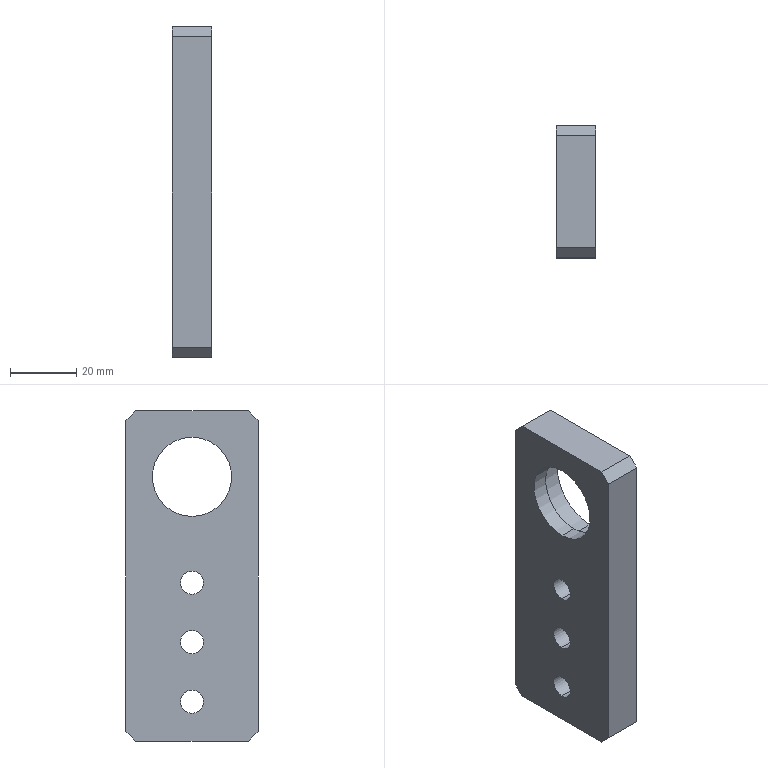Component | SolidWorks | ConveyorDriveWheelSidePlate-3 | 1 solid | 21 faces | box 12 x 40 x 100 mm | volume 39826 mm3 | plane 11 | cylinder 10 | commonest cylinder face diameters 7 x6 24 x2 28 x2 | material Plain Carbon Steel
build123d program:
from build123d import *

# Parameters (mm, degrees)
SKETCH1_W           = 100
SKETCH1_H           = 40
BOSS_EXTRUDE1_DEPTH = 12
SKETCH2_R           = 14
CUT_EXTRUDE1_DEPTH  = 7
SKETCH3_R           = 3.5
CUT_EXTRUDE2_DEPTH  = 56.172
SKETCH4_R           = 12
CUT_EXTRUDE3_DEPTH  = 55.305
CHAMFER1_SIZE       = 3


with BuildPart() as part:
    # Sketch1 → Boss-Extrude1 (new body)
    with BuildSketch(Plane(origin=(0, 0, 0), x_dir=(0, 0, -1), z_dir=(1, 0, 0))):
        Rectangle(SKETCH1_W, SKETCH1_H)
    extrude(amount=BOSS_EXTRUDE1_DEPTH)

    # Sketch2 → Cut-Extrude1 (cut)
    with BuildSketch(Plane(origin=(12, 0, 0), x_dir=(0, 0, -1), z_dir=(1, 0, 0))):
        with Locations((30, 0)):
            Circle(SKETCH2_R)
    extrude(amount=-CUT_EXTRUDE1_DEPTH, mode=Mode.SUBTRACT)

    # Sketch3 → Cut-Extrude2 (cut, through all)
    with BuildSketch(Plane.ZY):
        with Locations((38, 0)):
            Circle(SKETCH3_R)
        with Locations((2, 0)):
            Circle(SKETCH3_R)
        with Locations((20, 0)):
            Circle(SKETCH3_R)
    extrude(amount=-CUT_EXTRUDE2_DEPTH, mode=Mode.SUBTRACT)

    # Sketch4 → Cut-Extrude3 (cut, through all)
    with BuildSketch(Plane(origin=(5, 0, 0), x_dir=(0, 0, -1), z_dir=(1, 0, 0))):
        with Locations((30, 0)):
            Circle(SKETCH4_R)
    extrude(amount=-CUT_EXTRUDE3_DEPTH, mode=Mode.SUBTRACT)

    # Chamfer1
    chamfer1_edges = [part.edges().sort_by_distance(p)[0] for p in [
        (6, -20, -50),
        (6, -20, 50),
        (6, 20, 50),
        (6, 20, -50),
    ]]
    chamfer(chamfer1_edges, length=CHAMFER1_SIZE)


solid = part.part

# Placed as in the assembly
solid = solid.moved(Location((35.45, 5.646, 1505), (180, 0, 0)))
STEP:
#1=COLOUR_RGB('',0.7922,0.8196,0.9333);
#2=FILL_AREA_STYLE_COLOUR('',#1);
#3=FILL_AREA_STYLE('',(#2));
#4=SURFACE_STYLE_FILL_AREA(#3);
#5=SURFACE_SIDE_STYLE('',(#4));
#6=SURFACE_STYLE_USAGE(.BOTH.,#5);
#7=PRESENTATION_STYLE_ASSIGNMENT((#6));
#8=CARTESIAN_POINT('',(1.396,0.2223,59.961));
#9=VERTEX_POINT('',#8);
#10=CARTESIAN_POINT('',(1.396,0.2223,60.906));
#11=VERTEX_POINT('',#10);
#12=CARTESIAN_POINT('',(1.396,0.2223,60.433));
#13=DIRECTION('',(1.,-0.,-0.));
#14=DIRECTION('',(0.,0.,1.));
#15=AXIS2_PLACEMENT_3D('',#12,#13,#14);
#16=CIRCLE('',#15,0.4724);
#17=EDGE_CURVE('',#9,#11,#16,.T.);
#18=ORIENTED_EDGE('',*,*,#17,.F.);
#19=CARTESIAN_POINT('',(1.593,0.2223,59.961));
#20=VERTEX_POINT('',#19);
#21=CARTESIAN_POINT('',(1.396,0.2223,59.961));
#22=DIRECTION('',(1.,-0.,-0.));
#23=VECTOR('',#22,39.37);
#24=LINE('',#21,#23);
#25=EDGE_CURVE('',#9,#20,#24,.T.);
#26=ORIENTED_EDGE('',*,*,#25,.T.);
#27=CARTESIAN_POINT('',(1.593,0.2223,60.906));
#28=VERTEX_POINT('',#27);
#29=CARTESIAN_POINT('',(1.593,0.2223,60.433));
#30=DIRECTION('',(1.,-0.,-0.));
#31=DIRECTION('',(0.,0.,1.));
#32=AXIS2_PLACEMENT_3D('',#29,#30,#31);
#33=CIRCLE('',#32,0.4724);
#34=EDGE_CURVE('',#20,#28,#33,.T.);
#35=ORIENTED_EDGE('',*,*,#34,.T.);
#36=CARTESIAN_POINT('',(1.396,0.2223,60.906));
#37=DIRECTION('',(1.,-0.,-0.));
#38=VECTOR('',#37,39.37);
#39=LINE('',#36,#38);
#40=EDGE_CURVE('',#11,#28,#39,.T.);
#41=ORIENTED_EDGE('',*,*,#40,.F.);
#42=EDGE_LOOP('',(#18,#26,#35,#41));
#43=FACE_OUTER_BOUND('',#42,.T.);
#44=CARTESIAN_POINT('',(1.396,0.2223,60.433));
#45=DIRECTION('',(1.,-0.,-0.));
#46=DIRECTION('',(0.,0.,1.));
#47=AXIS2_PLACEMENT_3D('',#44,#45,#46);
#48=CYLINDRICAL_SURFACE('',#47,0.4724);
#49=ADVANCED_FACE('',(#43),#48,.F.);
#50=CARTESIAN_POINT('',(1.868,0.2223,58.602));
#51=VERTEX_POINT('',#50);
#52=CARTESIAN_POINT('',(1.868,0.2223,58.327));
#53=VERTEX_POINT('',#52);
#54=CARTESIAN_POINT('',(1.868,0.2223,58.465));
#55=DIRECTION('',(-1.,0.,0.));
#56=DIRECTION('',(0.,0.,-1.));
#57=AXIS2_PLACEMENT_3D('',#54,#55,#56);
#58=CIRCLE('',#57,0.1378);
#59=EDGE_CURVE('',#51,#53,#58,.T.);
#60=ORIENTED_EDGE('',*,*,#59,.F.);
#61=CARTESIAN_POINT('',(1.396,0.2223,58.602));
#62=VERTEX_POINT('',#61);
#63=CARTESIAN_POINT('',(1.868,0.2223,58.602));
#64=DIRECTION('',(-1.,0.,0.));
#65=VECTOR('',#64,39.37);
#66=LINE('',#63,#65);
#67=EDGE_CURVE('',#51,#62,#66,.T.);
#68=ORIENTED_EDGE('',*,*,#67,.T.);
#69=CARTESIAN_POINT('',(1.396,0.2223,58.327));
#70=VERTEX_POINT('',#69);
#71=CARTESIAN_POINT('',(1.396,0.2223,58.465));
#72=DIRECTION('',(-1.,0.,0.));
#73=DIRECTION('',(0.,0.,-1.));
#74=AXIS2_PLACEMENT_3D('',#71,#72,#73);
#75=CIRCLE('',#74,0.1378);
#76=EDGE_CURVE('',#62,#70,#75,.T.);
#77=ORIENTED_EDGE('',*,*,#76,.T.);
#78=CARTESIAN_POINT('',(1.868,0.2223,58.327));
#79=DIRECTION('',(-1.,0.,0.));
#80=VECTOR('',#79,39.37);
#81=LINE('',#78,#80);
#82=EDGE_CURVE('',#53,#70,#81,.T.);
#83=ORIENTED_EDGE('',*,*,#82,.F.);
#84=EDGE_LOOP('',(#60,#68,#77,#83));
#85=FACE_OUTER_BOUND('',#84,.T.);
#86=CARTESIAN_POINT('',(1.868,0.2223,58.465));
#87=DIRECTION('',(-1.,0.,0.));
#88=DIRECTION('',(0.,0.,-1.));
#89=AXIS2_PLACEMENT_3D('',#86,#87,#88);
#90=CYLINDRICAL_SURFACE('',#89,0.1378);
#91=ADVANCED_FACE('',(#85),#90,.F.);
#92=CARTESIAN_POINT('',(1.868,0.2223,59.311));
#93=VERTEX_POINT('',#92);
#94=CARTESIAN_POINT('',(1.868,0.2223,59.035));
#95=VERTEX_POINT('',#94);
#96=CARTESIAN_POINT('',(1.868,0.2223,59.173));
#97=DIRECTION('',(-1.,0.,0.));
#98=DIRECTION('',(0.,0.,-1.));
#99=AXIS2_PLACEMENT_3D('',#96,#97,#98);
#100=CIRCLE('',#99,0.1378);
#101=EDGE_CURVE('',#93,#95,#100,.T.);
#102=ORIENTED_EDGE('',*,*,#101,.F.);
#103=CARTESIAN_POINT('',(1.396,0.2223,59.311));
#104=VERTEX_POINT('',#103);
#105=CARTESIAN_POINT('',(1.868,0.2223,59.311));
#106=DIRECTION('',(-1.,0.,0.));
#107=VECTOR('',#106,39.37);
#108=LINE('',#105,#107);
#109=EDGE_CURVE('',#93,#104,#108,.T.);
#110=ORIENTED_EDGE('',*,*,#109,.T.);
#111=CARTESIAN_POINT('',(1.396,0.2223,59.035));
#112=VERTEX_POINT('',#111);
#113=CARTESIAN_POINT('',(1.396,0.2223,59.173));
#114=DIRECTION('',(-1.,0.,0.));
#115=DIRECTION('',(0.,0.,-1.));
#116=AXIS2_PLACEMENT_3D('',#113,#114,#115);
#117=CIRCLE('',#116,0.1378);
#118=EDGE_CURVE('',#104,#112,#117,.T.);
#119=ORIENTED_EDGE('',*,*,#118,.T.);
#120=CARTESIAN_POINT('',(1.868,0.2223,59.035));
#121=DIRECTION('',(-1.,0.,0.));
#122=VECTOR('',#121,39.37);
#123=LINE('',#120,#122);
#124=EDGE_CURVE('',#95,#112,#123,.T.);
#125=ORIENTED_EDGE('',*,*,#124,.F.);
#126=EDGE_LOOP('',(#102,#110,#119,#125));
#127=FACE_OUTER_BOUND('',#126,.T.);
#128=CARTESIAN_POINT('',(1.868,0.2223,59.173));
#129=DIRECTION('',(-1.,0.,0.));
#130=DIRECTION('',(0.,0.,-1.));
#131=AXIS2_PLACEMENT_3D('',#128,#129,#130);
#132=CYLINDRICAL_SURFACE('',#131,0.1378);
#133=ADVANCED_FACE('',(#127),#132,.F.);
#134=CARTESIAN_POINT('',(1.868,0.2223,57.894));
#135=VERTEX_POINT('',#134);
#136=CARTESIAN_POINT('',(1.868,0.2223,57.618));
#137=VERTEX_POINT('',#136);
#138=CARTESIAN_POINT('',(1.868,0.2223,57.756));
#139=DIRECTION('',(-1.,0.,0.));
#140=DIRECTION('',(0.,0.,-1.));
#141=AXIS2_PLACEMENT_3D('',#138,#139,#140);
#142=CIRCLE('',#141,0.1378);
#143=EDGE_CURVE('',#135,#137,#142,.T.);
#144=ORIENTED_EDGE('',*,*,#143,.F.);
#145=CARTESIAN_POINT('',(1.396,0.2223,57.894));
#146=VERTEX_POINT('',#145);
#147=CARTESIAN_POINT('',(1.868,0.2223,57.894));
#148=DIRECTION('',(-1.,0.,0.));
#149=VECTOR('',#148,39.37);
#150=LINE('',#147,#149);
#151=EDGE_CURVE('',#135,#146,#150,.T.);
#152=ORIENTED_EDGE('',*,*,#151,.T.);
#153=CARTESIAN_POINT('',(1.396,0.2223,57.618));
#154=VERTEX_POINT('',#153);
#155=CARTESIAN_POINT('',(1.396,0.2223,57.756));
#156=DIRECTION('',(-1.,0.,0.));
#157=DIRECTION('',(0.,0.,-1.));
#158=AXIS2_PLACEMENT_3D('',#155,#156,#157);
#159=CIRCLE('',#158,0.1378);
#160=EDGE_CURVE('',#146,#154,#159,.T.);
#161=ORIENTED_EDGE('',*,*,#160,.T.);
#162=CARTESIAN_POINT('',(1.868,0.2223,57.618));
#163=DIRECTION('',(-1.,0.,0.));
#164=VECTOR('',#163,39.37);
#165=LINE('',#162,#164);
#166=EDGE_CURVE('',#137,#154,#165,.T.);
#167=ORIENTED_EDGE('',*,*,#166,.F.);
#168=EDGE_LOOP('',(#144,#152,#161,#167));
#169=FACE_OUTER_BOUND('',#168,.T.);
#170=CARTESIAN_POINT('',(1.868,0.2223,57.756));
#171=DIRECTION('',(-1.,0.,0.));
#172=DIRECTION('',(0.,0.,-1.));
#173=AXIS2_PLACEMENT_3D('',#170,#171,#172);
#174=CYLINDRICAL_SURFACE('',#173,0.1378);
#175=ADVANCED_FACE('',(#169),#174,.F.);
#176=CARTESIAN_POINT('',(1.593,0.2223,59.882));
#177=VERTEX_POINT('',#176);
#178=CARTESIAN_POINT('',(1.593,0.2223,60.984));
#179=VERTEX_POINT('',#178);
#180=CARTESIAN_POINT('',(1.593,0.2223,60.433));
#181=DIRECTION('',(1.,-0.,-0.));
#182=DIRECTION('',(0.,0.,1.));
#183=AXIS2_PLACEMENT_3D('',#180,#181,#182);
#184=CIRCLE('',#183,0.5512);
#185=EDGE_CURVE('',#177,#179,#184,.T.);
#186=ORIENTED_EDGE('',*,*,#185,.F.);
#187=CARTESIAN_POINT('',(1.868,0.2223,59.882));
#188=VERTEX_POINT('',#187);
#189=CARTESIAN_POINT('',(1.593,0.2223,59.882));
#190=DIRECTION('',(1.,-0.,-0.));
#191=VECTOR('',#190,39.37);
#192=LINE('',#189,#191);
#193=EDGE_CURVE('',#177,#188,#192,.T.);
#194=ORIENTED_EDGE('',*,*,#193,.T.);
#195=CARTESIAN_POINT('',(1.868,0.2223,60.984));
#196=VERTEX_POINT('',#195);
#197=CARTESIAN_POINT('',(1.868,0.2223,60.433));
#198=DIRECTION('',(1.,-0.,-0.));
#199=DIRECTION('',(0.,0.,1.));
#200=AXIS2_PLACEMENT_3D('',#197,#198,#199);
#201=CIRCLE('',#200,0.5512);
#202=EDGE_CURVE('',#188,#196,#201,.T.);
#203=ORIENTED_EDGE('',*,*,#202,.T.);
#204=CARTESIAN_POINT('',(1.593,0.2223,60.984));
#205=DIRECTION('',(1.,-0.,-0.));
#206=VECTOR('',#205,39.37);
#207=LINE('',#204,#206);
#208=EDGE_CURVE('',#179,#196,#207,.T.);
#209=ORIENTED_EDGE('',*,*,#208,.F.);
#210=EDGE_LOOP('',(#186,#194,#203,#209));
#211=FACE_OUTER_BOUND('',#210,.T.);
#212=CARTESIAN_POINT('',(1.593,0.2223,60.433));
#213=DIRECTION('',(1.,-0.,-0.));
#214=DIRECTION('',(0.,0.,1.));
#215=AXIS2_PLACEMENT_3D('',#212,#213,#214);
#216=CYLINDRICAL_SURFACE('',#215,0.5512);
#217=ADVANCED_FACE('',(#211),#216,.F.);
#218=CARTESIAN_POINT('',(1.868,0.8916,61.22));
#219=VERTEX_POINT('',#218);
#220=CARTESIAN_POINT('',(1.868,-0.447,61.22));
#221=VERTEX_POINT('',#220);
#222=CARTESIAN_POINT('',(1.868,1.01,61.22));
#223=DIRECTION('',(-0.,-1.,0.));
#224=VECTOR('',#223,39.37);
#225=LINE('',#222,#224);
#226=EDGE_CURVE('',#219,#221,#225,.T.);
#227=ORIENTED_EDGE('',*,*,#226,.F.);
#228=CARTESIAN_POINT('',(1.396,0.8916,61.22));
#229=VERTEX_POINT('',#228);
#230=CARTESIAN_POINT('',(1.868,0.8916,61.22));
#231=DIRECTION('',(-1.,0.,0.));
#232=VECTOR('',#231,39.37);
#233=LINE('',#230,#232);
#234=EDGE_CURVE('',#219,#229,#233,.T.);
#235=ORIENTED_EDGE('',*,*,#234,.T.);
#236=CARTESIAN_POINT('',(1.396,-0.447,61.22));
#237=VERTEX_POINT('',#236);
#238=CARTESIAN_POINT('',(1.396,1.01,61.22));
#239=DIRECTION('',(-0.,-1.,0.));
#240=VECTOR('',#239,39.37);
#241=LINE('',#238,#240);
#242=EDGE_CURVE('',#229,#237,#241,.T.);
#243=ORIENTED_EDGE('',*,*,#242,.T.);
#244=CARTESIAN_POINT('',(1.868,-0.447,61.22));
#245=DIRECTION('',(1.,-0.,-0.));
#246=VECTOR('',#245,39.37);
#247=LINE('',#244,#246);
#248=EDGE_CURVE('',#237,#221,#247,.T.);
#249=ORIENTED_EDGE('',*,*,#248,.T.);
#250=EDGE_LOOP('',(#227,#235,#243,#249));
#251=FACE_OUTER_BOUND('',#250,.T.);
#252=CARTESIAN_POINT('',(1.868,1.01,61.22));
#253=DIRECTION('',(-0.,-0.,-1.));
#254=DIRECTION('',(1.,-0.,-0.));
#255=AXIS2_PLACEMENT_3D('',#252,#253,#254);
#256=PLANE('',#255);
#257=ADVANCED_FACE('',(#251),#256,.F.);
#258=CARTESIAN_POINT('',(1.868,-0.5651,61.102));
#259=VERTEX_POINT('',#258);
#260=CARTESIAN_POINT('',(1.868,-0.5651,57.402));
#261=VERTEX_POINT('',#260);
#262=CARTESIAN_POINT('',(1.868,-0.5651,57.283));
#263=DIRECTION('',(-0.,0.,-1.));
#264=VECTOR('',#263,39.37);
#265=LINE('',#262,#264);
#266=EDGE_CURVE('',#259,#261,#265,.T.);
#267=ORIENTED_EDGE('',*,*,#266,.F.);
#268=CARTESIAN_POINT('',(1.396,-0.5651,61.102));
#269=VERTEX_POINT('',#268);
#270=CARTESIAN_POINT('',(1.868,-0.5651,61.102));
#271=DIRECTION('',(-1.,0.,0.));
#272=VECTOR('',#271,39.37);
#273=LINE('',#270,#272);
#274=EDGE_CURVE('',#259,#269,#273,.T.);
#275=ORIENTED_EDGE('',*,*,#274,.T.);
#276=CARTESIAN_POINT('',(1.396,-0.5651,57.402));
#277=VERTEX_POINT('',#276);
#278=CARTESIAN_POINT('',(1.396,-0.5651,57.283));
#279=DIRECTION('',(-0.,0.,-1.));
#280=VECTOR('',#279,39.37);
#281=LINE('',#278,#280);
#282=EDGE_CURVE('',#269,#277,#281,.T.);
#283=ORIENTED_EDGE('',*,*,#282,.T.);
#284=CARTESIAN_POINT('',(1.868,-0.5651,57.402));
#285=DIRECTION('',(1.,-0.,-0.));
#286=VECTOR('',#285,39.37);
#287=LINE('',#284,#286);
#288=EDGE_CURVE('',#277,#261,#287,.T.);
#289=ORIENTED_EDGE('',*,*,#288,.T.);
#290=EDGE_LOOP('',(#267,#275,#283,#289));
#291=FACE_OUTER_BOUND('',#290,.T.);
#292=CARTESIAN_POINT('',(1.868,-0.5651,57.283));
#293=DIRECTION('',(0.,1.,-0.));
#294=DIRECTION('',(0.,0.,1.));
#295=AXIS2_PLACEMENT_3D('',#292,#293,#294);
#296=PLANE('',#295);
#297=ADVANCED_FACE('',(#291),#296,.F.);
#298=CARTESIAN_POINT('',(1.396,-0.447,57.283));
#299=VERTEX_POINT('',#298);
#300=CARTESIAN_POINT('',(1.396,0.8916,57.283));
#301=VERTEX_POINT('',#300);
#302=CARTESIAN_POINT('',(1.396,1.01,57.283));
#303=DIRECTION('',(0.,1.,-0.));
#304=VECTOR('',#303,39.37);
#305=LINE('',#302,#304);
#306=EDGE_CURVE('',#299,#301,#305,.T.);
#307=ORIENTED_EDGE('',*,*,#306,.T.);
#308=CARTESIAN_POINT('',(1.868,0.8916,57.283));
#309=VERTEX_POINT('',#308);
#310=CARTESIAN_POINT('',(1.868,0.8916,57.283));
#311=DIRECTION('',(1.,-0.,-0.));
#312=VECTOR('',#311,39.37);
#313=LINE('',#310,#312);
#314=EDGE_CURVE('',#301,#309,#313,.T.);
#315=ORIENTED_EDGE('',*,*,#314,.T.);
#316=CARTESIAN_POINT('',(1.868,-0.447,57.283));
#317=VERTEX_POINT('',#316);
#318=CARTESIAN_POINT('',(1.868,1.01,57.283));
#319=DIRECTION('',(0.,1.,-0.));
#320=VECTOR('',#319,39.37);
#321=LINE('',#318,#320);
#322=EDGE_CURVE('',#317,#309,#321,.T.);
#323=ORIENTED_EDGE('',*,*,#322,.F.);
#324=CARTESIAN_POINT('',(1.868,-0.447,57.283));
#325=DIRECTION('',(-1.,0.,0.));
#326=VECTOR('',#325,39.37);
#327=LINE('',#324,#326);
#328=EDGE_CURVE('',#317,#299,#327,.T.);
#329=ORIENTED_EDGE('',*,*,#328,.T.);
#330=EDGE_LOOP('',(#307,#315,#323,#329));
#331=FACE_OUTER_BOUND('',#330,.T.);
#332=CARTESIAN_POINT('',(1.868,1.01,57.283));
#333=DIRECTION('',(0.,0.,1.));
#334=DIRECTION('',(-1.,0.,0.));
#335=AXIS2_PLACEMENT_3D('',#332,#333,#334);
#336=PLANE('',#335);
#337=ADVANCED_FACE('',(#331),#336,.F.);
#338=CARTESIAN_POINT('',(1.396,1.01,57.402));
#339=VERTEX_POINT('',#338);
#340=CARTESIAN_POINT('',(1.396,1.01,61.102));
#341=VERTEX_POINT('',#340);
#342=CARTESIAN_POINT('',(1.396,1.01,57.283));
#343=DIRECTION('',(0.,0.,1.));
#344=VECTOR('',#343,39.37);
#345=LINE('',#342,#344);
#346=EDGE_CURVE('',#339,#341,#345,.T.);
#347=ORIENTED_EDGE('',*,*,#346,.T.);
#348=CARTESIAN_POINT('',(1.868,1.01,61.102));
#349=VERTEX_POINT('',#348);
#350=CARTESIAN_POINT('',(1.868,1.01,61.102));
#351=DIRECTION('',(1.,-0.,-0.));
#352=VECTOR('',#351,39.37);
#353=LINE('',#350,#352);
#354=EDGE_CURVE('',#341,#349,#353,.T.);
#355=ORIENTED_EDGE('',*,*,#354,.T.);
#356=CARTESIAN_POINT('',(1.868,1.01,57.402));
#357=VERTEX_POINT('',#356);
#358=CARTESIAN_POINT('',(1.868,1.01,57.283));
#359=DIRECTION('',(0.,0.,1.));
#360=VECTOR('',#359,39.37);
#361=LINE('',#358,#360);
#362=EDGE_CURVE('',#357,#349,#361,.T.);
#363=ORIENTED_EDGE('',*,*,#362,.F.);
#364=CARTESIAN_POINT('',(1.868,1.01,57.402));
#365=DIRECTION('',(-1.,0.,0.));
#366=VECTOR('',#365,39.37);
#367=LINE('',#364,#366);
#368=EDGE_CURVE('',#357,#339,#367,.T.);
#369=ORIENTED_EDGE('',*,*,#368,.T.);
#370=EDGE_LOOP('',(#347,#355,#363,#369));
#371=FACE_OUTER_BOUND('',#370,.T.);
#372=CARTESIAN_POINT('',(1.868,1.01,57.283));
#373=DIRECTION('',(-0.,-1.,0.));
#374=DIRECTION('',(-0.,0.,-1.));
#375=AXIS2_PLACEMENT_3D('',#372,#373,#374);
#376=PLANE('',#375);
#377=ADVANCED_FACE('',(#371),#376,.F.);
#378=CARTESIAN_POINT('',(1.868,0.2223,58.465));
#379=DIRECTION('',(-1.,0.,0.));
#380=DIRECTION('',(0.,0.,-1.));
#381=AXIS2_PLACEMENT_3D('',#378,#379,#380);
#382=CIRCLE('',#381,0.1378);
#383=EDGE_CURVE('',#53,#51,#382,.T.);
#384=ORIENTED_EDGE('',*,*,#383,.T.);
#385=ORIENTED_EDGE('',*,*,#59,.T.);
#386=EDGE_LOOP('',(#384,#385));
#387=FACE_BOUND('',#386,.T.);
#388=CARTESIAN_POINT('',(1.868,0.2223,59.173));
#389=DIRECTION('',(-1.,0.,0.));
#390=DIRECTION('',(0.,0.,-1.));
#391=AXIS2_PLACEMENT_3D('',#388,#389,#390);
#392=CIRCLE('',#391,0.1378);
#393=EDGE_CURVE('',#95,#93,#392,.T.);
#394=ORIENTED_EDGE('',*,*,#393,.T.);
#395=ORIENTED_EDGE('',*,*,#101,.T.);
#396=EDGE_LOOP('',(#394,#395));
#397=FACE_BOUND('',#396,.T.);
#398=CARTESIAN_POINT('',(1.868,0.2223,57.756));
#399=DIRECTION('',(-1.,0.,0.));
#400=DIRECTION('',(0.,0.,-1.));
#401=AXIS2_PLACEMENT_3D('',#398,#399,#400);
#402=CIRCLE('',#401,0.1378);
#403=EDGE_CURVE('',#137,#135,#402,.T.);
#404=ORIENTED_EDGE('',*,*,#403,.T.);
#405=ORIENTED_EDGE('',*,*,#143,.T.);
#406=EDGE_LOOP('',(#404,#405));
#407=FACE_BOUND('',#406,.T.);
#408=CARTESIAN_POINT('',(1.868,0.2223,60.433));
#409=DIRECTION('',(1.,-0.,-0.));
#410=DIRECTION('',(0.,0.,1.));
#411=AXIS2_PLACEMENT_3D('',#408,#409,#410);
#412=CIRCLE('',#411,0.5512);
#413=EDGE_CURVE('',#196,#188,#412,.T.);
#414=ORIENTED_EDGE('',*,*,#413,.F.);
#415=ORIENTED_EDGE('',*,*,#202,.F.);
#416=EDGE_LOOP('',(#414,#415));
#417=FACE_BOUND('',#416,.T.);
#418=ORIENTED_EDGE('',*,*,#362,.T.);
#419=CARTESIAN_POINT('',(1.868,0.8916,61.22));
#420=DIRECTION('',(-0.,-0.7071,0.7071));
#421=VECTOR('',#420,39.37);
#422=LINE('',#419,#421);
#423=EDGE_CURVE('',#349,#219,#422,.T.);
#424=ORIENTED_EDGE('',*,*,#423,.T.);
#425=ORIENTED_EDGE('',*,*,#226,.T.);
#426=CARTESIAN_POINT('',(1.868,-0.5651,61.102));
#427=DIRECTION('',(-0.,-0.7071,-0.7071));
#428=VECTOR('',#427,39.37);
#429=LINE('',#426,#428);
#430=EDGE_CURVE('',#221,#259,#429,.T.);
#431=ORIENTED_EDGE('',*,*,#430,.T.);
#432=ORIENTED_EDGE('',*,*,#266,.T.);
#433=CARTESIAN_POINT('',(1.868,-0.447,57.283));
#434=DIRECTION('',(0.,0.7071,-0.7071));
#435=VECTOR('',#434,39.37);
#436=LINE('',#433,#435);
#437=EDGE_CURVE('',#261,#317,#436,.T.);
#438=ORIENTED_EDGE('',*,*,#437,.T.);
#439=ORIENTED_EDGE('',*,*,#322,.T.);
#440=CARTESIAN_POINT('',(1.868,1.01,57.402));
#441=DIRECTION('',(0.,0.7071,0.7071));
#442=VECTOR('',#441,39.37);
#443=LINE('',#440,#442);
#444=EDGE_CURVE('',#309,#357,#443,.T.);
#445=ORIENTED_EDGE('',*,*,#444,.T.);
#446=EDGE_LOOP('',(#418,#424,#425,#431,#432,#438,#439,#445));
#447=FACE_OUTER_BOUND('',#446,.T.);
#448=CARTESIAN_POINT('',(1.868,0.2223,59.252));
#449=DIRECTION('',(-1.,0.,0.));
#450=DIRECTION('',(-0.,0.,-1.));
#451=AXIS2_PLACEMENT_3D('',#448,#449,#450);
#452=PLANE('',#451);
#453=ADVANCED_FACE('',(#387,#397,#407,#417,#447),#452,.F.);
#454=CARTESIAN_POINT('',(1.396,0.2223,60.433));
#455=DIRECTION('',(1.,-0.,-0.));
#456=DIRECTION('',(0.,0.,1.));
#457=AXIS2_PLACEMENT_3D('',#454,#455,#456);
#458=CIRCLE('',#457,0.4724);
#459=EDGE_CURVE('',#11,#9,#458,.T.);
#460=ORIENTED_EDGE('',*,*,#459,.T.);
#461=ORIENTED_EDGE('',*,*,#17,.T.);
#462=EDGE_LOOP('',(#460,#461));
#463=FACE_BOUND('',#462,.T.);
#464=CARTESIAN_POINT('',(1.396,0.2223,58.465));
#465=DIRECTION('',(-1.,0.,0.));
#466=DIRECTION('',(0.,0.,-1.));
#467=AXIS2_PLACEMENT_3D('',#464,#465,#466);
#468=CIRCLE('',#467,0.1378);
#469=EDGE_CURVE('',#70,#62,#468,.T.);
#470=ORIENTED_EDGE('',*,*,#469,.F.);
#471=ORIENTED_EDGE('',*,*,#76,.F.);
#472=EDGE_LOOP('',(#470,#471));
#473=FACE_BOUND('',#472,.T.);
#474=CARTESIAN_POINT('',(1.396,0.2223,59.173));
#475=DIRECTION('',(-1.,0.,0.));
#476=DIRECTION('',(0.,0.,-1.));
#477=AXIS2_PLACEMENT_3D('',#474,#475,#476);
#478=CIRCLE('',#477,0.1378);
#479=EDGE_CURVE('',#112,#104,#478,.T.);
#480=ORIENTED_EDGE('',*,*,#479,.F.);
#481=ORIENTED_EDGE('',*,*,#118,.F.);
#482=EDGE_LOOP('',(#480,#481));
#483=FACE_BOUND('',#482,.T.);
#484=CARTESIAN_POINT('',(1.396,0.2223,57.756));
#485=DIRECTION('',(-1.,0.,0.));
#486=DIRECTION('',(0.,0.,-1.));
#487=AXIS2_PLACEMENT_3D('',#484,#485,#486);
#488=CIRCLE('',#487,0.1378);
#489=EDGE_CURVE('',#154,#146,#488,.T.);
#490=ORIENTED_EDGE('',*,*,#489,.F.);
#491=ORIENTED_EDGE('',*,*,#160,.F.);
#492=EDGE_LOOP('',(#490,#491));
#493=FACE_BOUND('',#492,.T.);
#494=ORIENTED_EDGE('',*,*,#242,.F.);
#495=CARTESIAN_POINT('',(1.396,1.541,60.571));
#496=DIRECTION('',(0.,0.7071,-0.7071));
#497=VECTOR('',#496,39.37);
#498=LINE('',#495,#497);
#499=EDGE_CURVE('',#229,#341,#498,.T.);
#500=ORIENTED_EDGE('',*,*,#499,.T.);
#501=ORIENTED_EDGE('',*,*,#346,.F.);
#502=CARTESIAN_POINT('',(1.396,1.541,57.933));
#503=DIRECTION('',(-0.,-0.7071,-0.7071));
#504=VECTOR('',#503,39.37);
#505=LINE('',#502,#504);
#506=EDGE_CURVE('',#339,#301,#505,.T.);
#507=ORIENTED_EDGE('',*,*,#506,.T.);
#508=ORIENTED_EDGE('',*,*,#306,.F.);
#509=CARTESIAN_POINT('',(1.396,-1.097,57.933));
#510=DIRECTION('',(-0.,-0.7071,0.7071));
#511=VECTOR('',#510,39.37);
#512=LINE('',#509,#511);
#513=EDGE_CURVE('',#299,#277,#512,.T.);
#514=ORIENTED_EDGE('',*,*,#513,.T.);
#515=ORIENTED_EDGE('',*,*,#282,.F.);
#516=CARTESIAN_POINT('',(1.396,-1.097,60.571));
#517=DIRECTION('',(0.,0.7071,0.7071));
#518=VECTOR('',#517,39.37);
#519=LINE('',#516,#518);
#520=EDGE_CURVE('',#269,#237,#519,.T.);
#521=ORIENTED_EDGE('',*,*,#520,.T.);
#522=EDGE_LOOP('',(#494,#500,#501,#507,#508,#514,#515,#521));
#523=FACE_OUTER_BOUND('',#522,.T.);
#524=CARTESIAN_POINT('',(1.396,0.2223,59.252));
#525=DIRECTION('',(-1.,0.,0.));
#526=DIRECTION('',(-0.,0.,-1.));
#527=AXIS2_PLACEMENT_3D('',#524,#525,#526);
#528=PLANE('',#527);
#529=ADVANCED_FACE('',(#463,#473,#483,#493,#523),#528,.T.);
#530=ORIENTED_EDGE('',*,*,#193,.F.);
#531=CARTESIAN_POINT('',(1.593,0.2223,60.433));
#532=DIRECTION('',(1.,-0.,-0.));
#533=DIRECTION('',(0.,0.,1.));
#534=AXIS2_PLACEMENT_3D('',#531,#532,#533);
#535=CIRCLE('',#534,0.5512);
#536=EDGE_CURVE('',#179,#177,#535,.T.);
#537=ORIENTED_EDGE('',*,*,#536,.F.);
#538=ORIENTED_EDGE('',*,*,#208,.T.);
#539=ORIENTED_EDGE('',*,*,#413,.T.);
#540=EDGE_LOOP('',(#530,#537,#538,#539));
#541=FACE_OUTER_BOUND('',#540,.T.);
#542=CARTESIAN_POINT('',(1.593,0.2223,60.433));
#543=DIRECTION('',(1.,-0.,-0.));
#544=DIRECTION('',(0.,0.,1.));
#545=AXIS2_PLACEMENT_3D('',#542,#543,#544);
#546=CYLINDRICAL_SURFACE('',#545,0.5512);
#547=ADVANCED_FACE('',(#541),#546,.F.);
#548=CARTESIAN_POINT('',(1.593,0.2223,60.433));
#549=DIRECTION('',(1.,-0.,-0.));
#550=DIRECTION('',(0.,0.,1.));
#551=AXIS2_PLACEMENT_3D('',#548,#549,#550);
#552=CIRCLE('',#551,0.4724);
#553=EDGE_CURVE('',#28,#20,#552,.T.);
#554=ORIENTED_EDGE('',*,*,#553,.F.);
#555=ORIENTED_EDGE('',*,*,#34,.F.);
#556=EDGE_LOOP('',(#554,#555));
#557=FACE_BOUND('',#556,.T.);
#558=ORIENTED_EDGE('',*,*,#536,.T.);
#559=ORIENTED_EDGE('',*,*,#185,.T.);
#560=EDGE_LOOP('',(#558,#559));
#561=FACE_OUTER_BOUND('',#560,.T.);
#562=CARTESIAN_POINT('',(1.593,0.2223,60.433));
#563=DIRECTION('',(1.,-0.,-0.));
#564=DIRECTION('',(0.,0.,1.));
#565=AXIS2_PLACEMENT_3D('',#562,#563,#564);
#566=PLANE('',#565);
#567=ADVANCED_FACE('',(#557,#561),#566,.T.);
#568=ORIENTED_EDGE('',*,*,#151,.F.);
#569=ORIENTED_EDGE('',*,*,#403,.F.);
#570=ORIENTED_EDGE('',*,*,#166,.T.);
#571=ORIENTED_EDGE('',*,*,#489,.T.);
#572=EDGE_LOOP('',(#568,#569,#570,#571));
#573=FACE_OUTER_BOUND('',#572,.T.);
#574=CARTESIAN_POINT('',(1.868,0.2223,57.756));
#575=DIRECTION('',(-1.,0.,0.));
#576=DIRECTION('',(0.,0.,-1.));
#577=AXIS2_PLACEMENT_3D('',#574,#575,#576);
#578=CYLINDRICAL_SURFACE('',#577,0.1378);
#579=ADVANCED_FACE('',(#573),#578,.F.);
#580=ORIENTED_EDGE('',*,*,#109,.F.);
#581=ORIENTED_EDGE('',*,*,#393,.F.);
#582=ORIENTED_EDGE('',*,*,#124,.T.);
#583=ORIENTED_EDGE('',*,*,#479,.T.);
#584=EDGE_LOOP('',(#580,#581,#582,#583));
#585=FACE_OUTER_BOUND('',#584,.T.);
#586=CARTESIAN_POINT('',(1.868,0.2223,59.173));
#587=DIRECTION('',(-1.,0.,0.));
#588=DIRECTION('',(0.,0.,-1.));
#589=AXIS2_PLACEMENT_3D('',#586,#587,#588);
#590=CYLINDRICAL_SURFACE('',#589,0.1378);
#591=ADVANCED_FACE('',(#585),#590,.F.);
#592=ORIENTED_EDGE('',*,*,#67,.F.);
#593=ORIENTED_EDGE('',*,*,#383,.F.);
#594=ORIENTED_EDGE('',*,*,#82,.T.);
#595=ORIENTED_EDGE('',*,*,#469,.T.);
#596=EDGE_LOOP('',(#592,#593,#594,#595));
#597=FACE_OUTER_BOUND('',#596,.T.);
#598=CARTESIAN_POINT('',(1.868,0.2223,58.465));
#599=DIRECTION('',(-1.,0.,0.));
#600=DIRECTION('',(0.,0.,-1.));
#601=AXIS2_PLACEMENT_3D('',#598,#599,#600);
#602=CYLINDRICAL_SURFACE('',#601,0.1378);
#603=ADVANCED_FACE('',(#597),#602,.F.);
#604=ORIENTED_EDGE('',*,*,#25,.F.);
#605=ORIENTED_EDGE('',*,*,#459,.F.);
#606=ORIENTED_EDGE('',*,*,#40,.T.);
#607=ORIENTED_EDGE('',*,*,#553,.T.);
#608=EDGE_LOOP('',(#604,#605,#606,#607));
#609=FACE_OUTER_BOUND('',#608,.T.);
#610=CARTESIAN_POINT('',(1.396,0.2223,60.433));
#611=DIRECTION('',(1.,-0.,-0.));
#612=DIRECTION('',(0.,0.,1.));
#613=AXIS2_PLACEMENT_3D('',#610,#611,#612);
#614=CYLINDRICAL_SURFACE('',#613,0.4724);
#615=ADVANCED_FACE('',(#609),#614,.F.);
#616=ORIENTED_EDGE('',*,*,#423,.F.);
#617=ORIENTED_EDGE('',*,*,#354,.F.);
#618=ORIENTED_EDGE('',*,*,#499,.F.);
#619=ORIENTED_EDGE('',*,*,#234,.F.);
#620=EDGE_LOOP('',(#616,#617,#618,#619));
#621=FACE_OUTER_BOUND('',#620,.T.);
#622=CARTESIAN_POINT('',(1.868,0.8916,61.22));
#623=DIRECTION('',(-0.,-0.7071,-0.7071));
#624=DIRECTION('',(-1.,0.,0.));
#625=AXIS2_PLACEMENT_3D('',#622,#623,#624);
#626=PLANE('',#625);
#627=ADVANCED_FACE('',(#621),#626,.F.);
#628=ORIENTED_EDGE('',*,*,#430,.F.);
#629=ORIENTED_EDGE('',*,*,#248,.F.);
#630=ORIENTED_EDGE('',*,*,#520,.F.);
#631=ORIENTED_EDGE('',*,*,#274,.F.);
#632=EDGE_LOOP('',(#628,#629,#630,#631));
#633=FACE_OUTER_BOUND('',#632,.T.);
#634=CARTESIAN_POINT('',(1.868,-0.5651,61.102));
#635=DIRECTION('',(0.,0.7071,-0.7071));
#636=DIRECTION('',(-1.,0.,0.));
#637=AXIS2_PLACEMENT_3D('',#634,#635,#636);
#638=PLANE('',#637);
#639=ADVANCED_FACE('',(#633),#638,.F.);
#640=ORIENTED_EDGE('',*,*,#444,.F.);
#641=ORIENTED_EDGE('',*,*,#314,.F.);
#642=ORIENTED_EDGE('',*,*,#506,.F.);
#643=ORIENTED_EDGE('',*,*,#368,.F.);
#644=EDGE_LOOP('',(#640,#641,#642,#643));
#645=FACE_OUTER_BOUND('',#644,.T.);
#646=CARTESIAN_POINT('',(1.868,1.01,57.402));
#647=DIRECTION('',(-0.,-0.7071,0.7071));
#648=DIRECTION('',(-1.,0.,0.));
#649=AXIS2_PLACEMENT_3D('',#646,#647,#648);
#650=PLANE('',#649);
#651=ADVANCED_FACE('',(#645),#650,.F.);
#652=ORIENTED_EDGE('',*,*,#437,.F.);
#653=ORIENTED_EDGE('',*,*,#288,.F.);
#654=ORIENTED_EDGE('',*,*,#513,.F.);
#655=ORIENTED_EDGE('',*,*,#328,.F.);
#656=EDGE_LOOP('',(#652,#653,#654,#655));
#657=FACE_OUTER_BOUND('',#656,.T.);
#658=CARTESIAN_POINT('',(1.868,-0.447,57.283));
#659=DIRECTION('',(0.,0.7071,0.7071));
#660=DIRECTION('',(-1.,0.,0.));
#661=AXIS2_PLACEMENT_3D('',#658,#659,#660);
#662=PLANE('',#661);
#663=ADVANCED_FACE('',(#657),#662,.F.);
#664=CLOSED_SHELL('',(#49,#91,#133,#175,#217,#257,#297,#337,#377,#453,#529,#547,#567,#579,#591,#603,#615,#627,#639,#651,#663));
#665=MANIFOLD_SOLID_BREP('',#664);
#666=STYLED_ITEM('',(#7),#665);
#667=PRESENTATION_LAYER_ASSIGNMENT('','',(#666));
#668=(LENGTH_UNIT()NAMED_UNIT(*)SI_UNIT($,.METRE.));
#669=LENGTH_MEASURE_WITH_UNIT(LENGTH_MEASURE(0.0254),#668);
#670=DIMENSIONAL_EXPONENTS(1.,0.,0.,0.,0.,0.,0.);
#671=(CONVERSION_BASED_UNIT('',#669)LENGTH_UNIT()NAMED_UNIT(#670));
#672=UNCERTAINTY_MEASURE_WITH_UNIT(LENGTH_MEASURE(0.00001),#671,'','');
#673=(NAMED_UNIT(*)PLANE_ANGLE_UNIT()SI_UNIT($,.RADIAN.));
#674=(NAMED_UNIT(*)SI_UNIT($,.STERADIAN.)SOLID_ANGLE_UNIT());
#675=(GEOMETRIC_REPRESENTATION_CONTEXT(3)GLOBAL_UNCERTAINTY_ASSIGNED_CONTEXT((#672))GLOBAL_UNIT_ASSIGNED_CONTEXT((#671,#673,#674))REPRESENTATION_CONTEXT('',''));
#676=MECHANICAL_DESIGN_GEOMETRIC_PRESENTATION_REPRESENTATION('',(#666),#675);
#677=CARTESIAN_POINT('',(0.,0.,0.));
#678=DIRECTION('',(0.,0.,1.));
#679=DIRECTION('',(1.,0.,0.));
#680=AXIS2_PLACEMENT_3D('',#677,#678,#679);
#681=(LENGTH_UNIT()NAMED_UNIT(*)SI_UNIT($,.METRE.));
#682=LENGTH_MEASURE_WITH_UNIT(LENGTH_MEASURE(0.0254),#681);
#683=DIMENSIONAL_EXPONENTS(1.,0.,0.,0.,0.,0.,0.);
#684=(CONVERSION_BASED_UNIT('',#682)LENGTH_UNIT()NAMED_UNIT(#683));
#685=UNCERTAINTY_MEASURE_WITH_UNIT(LENGTH_MEASURE(0.00001),#684,'','');
#686=(NAMED_UNIT(*)PLANE_ANGLE_UNIT()SI_UNIT($,.RADIAN.));
#687=(NAMED_UNIT(*)SI_UNIT($,.STERADIAN.)SOLID_ANGLE_UNIT());
#688=(GEOMETRIC_REPRESENTATION_CONTEXT(3)GLOBAL_UNCERTAINTY_ASSIGNED_CONTEXT((#685))GLOBAL_UNIT_ASSIGNED_CONTEXT((#684,#686,#687))REPRESENTATION_CONTEXT('',''));
#689=ADVANCED_BREP_SHAPE_REPRESENTATION('',(#665,#680),#688);